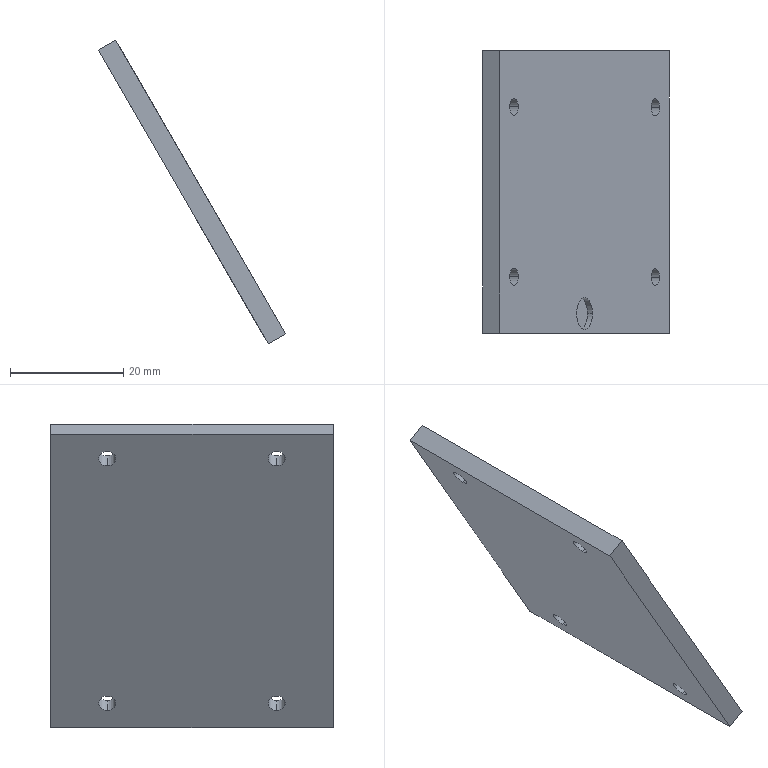Component | SolidWorks | LaserWorkingHeadCover(Upper)2-7 | 1 solid | 17 faces | box 33.03 x 50 x 53.71 mm | volume 10376 mm3 | cylinder 10 | plane 7 | commonest cylinder face diameters 3 x8 5.6 x2
build123d program:
from build123d import *

# Parameters (mm, degrees)
SKETCH1_2_W         = 60
SKETCH1_2_H         = 50
SKETCH1_2_R         = 1.5
BOSS_EXTRUDE1_DEPTH = 3.5
SKETCH1_R           = 2.8
CUT_EXTRUDE1_DEPTH  = 1


with BuildPart() as part:
    # Sketch1_2 → Boss-Extrude1 (new body)
    with BuildSketch(Plane.XY):
        Rectangle(SKETCH1_2_W, SKETCH1_2_H)
        with Locations((-25, 15)):
            Circle(SKETCH1_2_R, mode=Mode.SUBTRACT)
        with Locations((25, 15)):
            Circle(SKETCH1_2_R, mode=Mode.SUBTRACT)
        with Locations((25, -15)):
            Circle(SKETCH1_2_R, mode=Mode.SUBTRACT)
        with Locations((-25, -15)):
            Circle(SKETCH1_2_R, mode=Mode.SUBTRACT)
    extrude(amount=BOSS_EXTRUDE1_DEPTH)

    # Sketch1 → Cut-Extrude1 (cut)
    with BuildSketch(Plane(origin=(0, 0, 0), x_dir=(-1, 0, 0), z_dir=(0, 0, -1))):
        with Locations((0, -21.5)):
            Circle(SKETCH1_R)
    extrude(amount=-CUT_EXTRUDE1_DEPTH, mode=Mode.SUBTRACT)


solid = part.part

# Placed as in the assembly
solid = solid.moved(Location((-85.655, 40.506, 114), (-180, -60, 180)))
STEP:
#1=CARTESIAN_POINT('',(-3.461,0.7483,4.564));
#2=VERTEX_POINT('',#1);
#3=CARTESIAN_POINT('',(-3.351,0.7483,4.373));
#4=VERTEX_POINT('',#3);
#5=CARTESIAN_POINT('',(-3.406,0.7483,4.469));
#6=DIRECTION('',(0.866,-0.,0.5));
#7=DIRECTION('',(0.5,0.,-0.866));
#8=AXIS2_PLACEMENT_3D('',#5,#6,#7);
#9=CIRCLE('',#8,0.1102);
#10=EDGE_CURVE('',#2,#4,#9,.T.);
#11=ORIENTED_EDGE('',*,*,#10,.F.);
#12=CARTESIAN_POINT('',(-3.427,0.7483,4.584));
#13=VERTEX_POINT('',#12);
#14=CARTESIAN_POINT('',(-3.461,0.7483,4.564));
#15=DIRECTION('',(0.866,-0.,0.5));
#16=VECTOR('',#15,39.37);
#17=LINE('',#14,#16);
#18=EDGE_CURVE('',#2,#13,#17,.T.);
#19=ORIENTED_EDGE('',*,*,#18,.T.);
#20=CARTESIAN_POINT('',(-3.317,0.7483,4.393));
#21=VERTEX_POINT('',#20);
#22=CARTESIAN_POINT('',(-3.372,0.7483,4.488));
#23=DIRECTION('',(0.866,-0.,0.5));
#24=DIRECTION('',(0.5,0.,-0.866));
#25=AXIS2_PLACEMENT_3D('',#22,#23,#24);
#26=CIRCLE('',#25,0.1102);
#27=EDGE_CURVE('',#13,#21,#26,.T.);
#28=ORIENTED_EDGE('',*,*,#27,.T.);
#29=CARTESIAN_POINT('',(-3.351,0.7483,4.373));
#30=DIRECTION('',(0.866,-0.,0.5));
#31=VECTOR('',#30,39.37);
#32=LINE('',#29,#31);
#33=EDGE_CURVE('',#4,#21,#32,.T.);
#34=ORIENTED_EDGE('',*,*,#33,.F.);
#35=EDGE_LOOP('',(#11,#19,#28,#34));
#36=FACE_OUTER_BOUND('',#35,.T.);
#37=CARTESIAN_POINT('',(-3.406,0.7483,4.469));
#38=DIRECTION('',(0.866,-0.,0.5));
#39=DIRECTION('',(0.5,0.,-0.866));
#40=AXIS2_PLACEMENT_3D('',#37,#38,#39);
#41=CYLINDRICAL_SURFACE('',#40,0.1102);
#42=ADVANCED_FACE('',(#36),#41,.F.);
#43=CARTESIAN_POINT('',(-2.97,1.004,3.516));
#44=VERTEX_POINT('',#43);
#45=CARTESIAN_POINT('',(-3.029,1.004,3.618));
#46=VERTEX_POINT('',#45);
#47=CARTESIAN_POINT('',(-2.999,1.004,3.567));
#48=DIRECTION('',(-0.866,0.,-0.5));
#49=DIRECTION('',(-0.5,0.,0.866));
#50=AXIS2_PLACEMENT_3D('',#47,#48,#49);
#51=CIRCLE('',#50,0.05906);
#52=EDGE_CURVE('',#44,#46,#51,.T.);
#53=ORIENTED_EDGE('',*,*,#52,.T.);
#54=CARTESIAN_POINT('',(-2.91,1.004,3.687));
#55=VERTEX_POINT('',#54);
#56=CARTESIAN_POINT('',(-3.029,1.004,3.618));
#57=DIRECTION('',(0.866,-0.,0.5));
#58=VECTOR('',#57,39.37);
#59=LINE('',#56,#58);
#60=EDGE_CURVE('',#46,#55,#59,.T.);
#61=ORIENTED_EDGE('',*,*,#60,.T.);
#62=CARTESIAN_POINT('',(-2.851,1.004,3.585));
#63=VERTEX_POINT('',#62);
#64=CARTESIAN_POINT('',(-2.88,1.004,3.636));
#65=DIRECTION('',(-0.866,0.,-0.5));
#66=DIRECTION('',(-0.5,0.,0.866));
#67=AXIS2_PLACEMENT_3D('',#64,#65,#66);
#68=CIRCLE('',#67,0.05906);
#69=EDGE_CURVE('',#63,#55,#68,.T.);
#70=ORIENTED_EDGE('',*,*,#69,.F.);
#71=CARTESIAN_POINT('',(-2.97,1.004,3.516));
#72=DIRECTION('',(0.866,-0.,0.5));
#73=VECTOR('',#72,39.37);
#74=LINE('',#71,#73);
#75=EDGE_CURVE('',#44,#63,#74,.T.);
#76=ORIENTED_EDGE('',*,*,#75,.F.);
#77=EDGE_LOOP('',(#53,#61,#70,#76));
#78=FACE_OUTER_BOUND('',#77,.T.);
#79=CARTESIAN_POINT('',(-2.999,1.004,3.567));
#80=DIRECTION('',(0.866,-0.,0.5));
#81=DIRECTION('',(0.5,0.,-0.866));
#82=AXIS2_PLACEMENT_3D('',#79,#80,#81);
#83=CYLINDRICAL_SURFACE('',#82,0.05906);
#84=ADVANCED_FACE('',(#78),#83,.F.);
#85=CARTESIAN_POINT('',(-3.954,1.004,5.221));
#86=VERTEX_POINT('',#85);
#87=CARTESIAN_POINT('',(-4.013,1.004,5.323));
#88=VERTEX_POINT('',#87);
#89=CARTESIAN_POINT('',(-3.984,1.004,5.272));
#90=DIRECTION('',(-0.866,0.,-0.5));
#91=DIRECTION('',(-0.5,0.,0.866));
#92=AXIS2_PLACEMENT_3D('',#89,#90,#91);
#93=CIRCLE('',#92,0.05906);
#94=EDGE_CURVE('',#86,#88,#93,.T.);
#95=ORIENTED_EDGE('',*,*,#94,.T.);
#96=CARTESIAN_POINT('',(-3.894,1.004,5.392));
#97=VERTEX_POINT('',#96);
#98=CARTESIAN_POINT('',(-4.013,1.004,5.323));
#99=DIRECTION('',(0.866,-0.,0.5));
#100=VECTOR('',#99,39.37);
#101=LINE('',#98,#100);
#102=EDGE_CURVE('',#88,#97,#101,.T.);
#103=ORIENTED_EDGE('',*,*,#102,.T.);
#104=CARTESIAN_POINT('',(-3.835,1.004,5.289));
#105=VERTEX_POINT('',#104);
#106=CARTESIAN_POINT('',(-3.864,1.004,5.341));
#107=DIRECTION('',(-0.866,0.,-0.5));
#108=DIRECTION('',(-0.5,0.,0.866));
#109=AXIS2_PLACEMENT_3D('',#106,#107,#108);
#110=CIRCLE('',#109,0.05906);
#111=EDGE_CURVE('',#105,#97,#110,.T.);
#112=ORIENTED_EDGE('',*,*,#111,.F.);
#113=CARTESIAN_POINT('',(-3.954,1.004,5.221));
#114=DIRECTION('',(0.866,-0.,0.5));
#115=VECTOR('',#114,39.37);
#116=LINE('',#113,#115);
#117=EDGE_CURVE('',#86,#105,#116,.T.);
#118=ORIENTED_EDGE('',*,*,#117,.F.);
#119=EDGE_LOOP('',(#95,#103,#112,#118));
#120=FACE_OUTER_BOUND('',#119,.T.);
#121=CARTESIAN_POINT('',(-3.984,1.004,5.272));
#122=DIRECTION('',(0.866,-0.,0.5));
#123=DIRECTION('',(0.5,0.,-0.866));
#124=AXIS2_PLACEMENT_3D('',#121,#122,#123);
#125=CYLINDRICAL_SURFACE('',#124,0.05906);
#126=ADVANCED_FACE('',(#120),#125,.F.);
#127=CARTESIAN_POINT('',(-3.954,2.185,5.221));
#128=VERTEX_POINT('',#127);
#129=CARTESIAN_POINT('',(-4.013,2.185,5.323));
#130=VERTEX_POINT('',#129);
#131=CARTESIAN_POINT('',(-3.984,2.185,5.272));
#132=DIRECTION('',(-0.866,0.,-0.5));
#133=DIRECTION('',(-0.5,0.,0.866));
#134=AXIS2_PLACEMENT_3D('',#131,#132,#133);
#135=CIRCLE('',#134,0.05906);
#136=EDGE_CURVE('',#128,#130,#135,.T.);
#137=ORIENTED_EDGE('',*,*,#136,.T.);
#138=CARTESIAN_POINT('',(-3.894,2.185,5.392));
#139=VERTEX_POINT('',#138);
#140=CARTESIAN_POINT('',(-4.013,2.185,5.323));
#141=DIRECTION('',(0.866,-0.,0.5));
#142=VECTOR('',#141,39.37);
#143=LINE('',#140,#142);
#144=EDGE_CURVE('',#130,#139,#143,.T.);
#145=ORIENTED_EDGE('',*,*,#144,.T.);
#146=CARTESIAN_POINT('',(-3.835,2.185,5.289));
#147=VERTEX_POINT('',#146);
#148=CARTESIAN_POINT('',(-3.864,2.185,5.341));
#149=DIRECTION('',(-0.866,0.,-0.5));
#150=DIRECTION('',(-0.5,0.,0.866));
#151=AXIS2_PLACEMENT_3D('',#148,#149,#150);
#152=CIRCLE('',#151,0.05906);
#153=EDGE_CURVE('',#147,#139,#152,.T.);
#154=ORIENTED_EDGE('',*,*,#153,.F.);
#155=CARTESIAN_POINT('',(-3.954,2.185,5.221));
#156=DIRECTION('',(0.866,-0.,0.5));
#157=VECTOR('',#156,39.37);
#158=LINE('',#155,#157);
#159=EDGE_CURVE('',#128,#147,#158,.T.);
#160=ORIENTED_EDGE('',*,*,#159,.F.);
#161=EDGE_LOOP('',(#137,#145,#154,#160));
#162=FACE_OUTER_BOUND('',#161,.T.);
#163=CARTESIAN_POINT('',(-3.984,2.185,5.272));
#164=DIRECTION('',(0.866,-0.,0.5));
#165=DIRECTION('',(0.5,0.,-0.866));
#166=AXIS2_PLACEMENT_3D('',#163,#164,#165);
#167=CYLINDRICAL_SURFACE('',#166,0.05906);
#168=ADVANCED_FACE('',(#162),#167,.F.);
#169=CARTESIAN_POINT('',(-2.97,2.185,3.516));
#170=VERTEX_POINT('',#169);
#171=CARTESIAN_POINT('',(-3.029,2.185,3.618));
#172=VERTEX_POINT('',#171);
#173=CARTESIAN_POINT('',(-2.999,2.185,3.567));
#174=DIRECTION('',(-0.866,0.,-0.5));
#175=DIRECTION('',(-0.5,0.,0.866));
#176=AXIS2_PLACEMENT_3D('',#173,#174,#175);
#177=CIRCLE('',#176,0.05906);
#178=EDGE_CURVE('',#170,#172,#177,.T.);
#179=ORIENTED_EDGE('',*,*,#178,.T.);
#180=CARTESIAN_POINT('',(-2.91,2.185,3.687));
#181=VERTEX_POINT('',#180);
#182=CARTESIAN_POINT('',(-3.029,2.185,3.618));
#183=DIRECTION('',(0.866,-0.,0.5));
#184=VECTOR('',#183,39.37);
#185=LINE('',#182,#184);
#186=EDGE_CURVE('',#172,#181,#185,.T.);
#187=ORIENTED_EDGE('',*,*,#186,.T.);
#188=CARTESIAN_POINT('',(-2.851,2.185,3.585));
#189=VERTEX_POINT('',#188);
#190=CARTESIAN_POINT('',(-2.88,2.185,3.636));
#191=DIRECTION('',(-0.866,0.,-0.5));
#192=DIRECTION('',(-0.5,0.,0.866));
#193=AXIS2_PLACEMENT_3D('',#190,#191,#192);
#194=CIRCLE('',#193,0.05906);
#195=EDGE_CURVE('',#189,#181,#194,.T.);
#196=ORIENTED_EDGE('',*,*,#195,.F.);
#197=CARTESIAN_POINT('',(-2.97,2.185,3.516));
#198=DIRECTION('',(0.866,-0.,0.5));
#199=VECTOR('',#198,39.37);
#200=LINE('',#197,#199);
#201=EDGE_CURVE('',#170,#189,#200,.T.);
#202=ORIENTED_EDGE('',*,*,#201,.F.);
#203=EDGE_LOOP('',(#179,#187,#196,#202));
#204=FACE_OUTER_BOUND('',#203,.T.);
#205=CARTESIAN_POINT('',(-2.999,2.185,3.567));
#206=DIRECTION('',(0.866,-0.,0.5));
#207=DIRECTION('',(0.5,0.,-0.866));
#208=AXIS2_PLACEMENT_3D('',#205,#206,#207);
#209=CYLINDRICAL_SURFACE('',#208,0.05906);
#210=ADVANCED_FACE('',(#204),#209,.F.);
#211=ORIENTED_EDGE('',*,*,#94,.F.);
#212=CARTESIAN_POINT('',(-3.984,1.004,5.272));
#213=DIRECTION('',(-0.866,0.,-0.5));
#214=DIRECTION('',(-0.5,0.,0.866));
#215=AXIS2_PLACEMENT_3D('',#212,#213,#214);
#216=CIRCLE('',#215,0.05906);
#217=EDGE_CURVE('',#88,#86,#216,.T.);
#218=ORIENTED_EDGE('',*,*,#217,.F.);
#219=EDGE_LOOP('',(#211,#218));
#220=FACE_BOUND('',#219,.T.);
#221=ORIENTED_EDGE('',*,*,#178,.F.);
#222=CARTESIAN_POINT('',(-2.999,2.185,3.567));
#223=DIRECTION('',(-0.866,0.,-0.5));
#224=DIRECTION('',(-0.5,0.,0.866));
#225=AXIS2_PLACEMENT_3D('',#222,#223,#224);
#226=CIRCLE('',#225,0.05906);
#227=EDGE_CURVE('',#172,#170,#226,.T.);
#228=ORIENTED_EDGE('',*,*,#227,.F.);
#229=EDGE_LOOP('',(#221,#228));
#230=FACE_BOUND('',#229,.T.);
#231=CARTESIAN_POINT('',(-4.082,0.6105,5.442));
#232=VERTEX_POINT('',#231);
#233=CARTESIAN_POINT('',(-4.082,2.579,5.442));
#234=VERTEX_POINT('',#233);
#235=CARTESIAN_POINT('',(-4.082,2.579,5.442));
#236=DIRECTION('',(0.,1.,-0.));
#237=VECTOR('',#236,39.37);
#238=LINE('',#235,#237);
#239=EDGE_CURVE('',#232,#234,#238,.T.);
#240=ORIENTED_EDGE('',*,*,#239,.T.);
#241=CARTESIAN_POINT('',(-2.901,2.579,3.396));
#242=VERTEX_POINT('',#241);
#243=CARTESIAN_POINT('',(-2.901,2.579,3.396));
#244=DIRECTION('',(0.5,-0.,-0.866));
#245=VECTOR('',#244,39.37);
#246=LINE('',#243,#245);
#247=EDGE_CURVE('',#234,#242,#246,.T.);
#248=ORIENTED_EDGE('',*,*,#247,.T.);
#249=CARTESIAN_POINT('',(-2.901,0.6105,3.396));
#250=VERTEX_POINT('',#249);
#251=CARTESIAN_POINT('',(-2.901,2.579,3.396));
#252=DIRECTION('',(-0.,-1.,0.));
#253=VECTOR('',#252,39.37);
#254=LINE('',#251,#253);
#255=EDGE_CURVE('',#242,#250,#254,.T.);
#256=ORIENTED_EDGE('',*,*,#255,.T.);
#257=CARTESIAN_POINT('',(-2.901,0.6105,3.396));
#258=DIRECTION('',(-0.5,0.,0.866));
#259=VECTOR('',#258,39.37);
#260=LINE('',#257,#259);
#261=EDGE_CURVE('',#250,#232,#260,.T.);
#262=ORIENTED_EDGE('',*,*,#261,.T.);
#263=EDGE_LOOP('',(#240,#248,#256,#262));
#264=FACE_OUTER_BOUND('',#263,.T.);
#265=ORIENTED_EDGE('',*,*,#136,.F.);
#266=CARTESIAN_POINT('',(-3.984,2.185,5.272));
#267=DIRECTION('',(-0.866,0.,-0.5));
#268=DIRECTION('',(-0.5,0.,0.866));
#269=AXIS2_PLACEMENT_3D('',#266,#267,#268);
#270=CIRCLE('',#269,0.05906);
#271=EDGE_CURVE('',#130,#128,#270,.T.);
#272=ORIENTED_EDGE('',*,*,#271,.F.);
#273=EDGE_LOOP('',(#265,#272));
#274=FACE_BOUND('',#273,.T.);
#275=ORIENTED_EDGE('',*,*,#52,.F.);
#276=CARTESIAN_POINT('',(-2.999,1.004,3.567));
#277=DIRECTION('',(-0.866,0.,-0.5));
#278=DIRECTION('',(-0.5,0.,0.866));
#279=AXIS2_PLACEMENT_3D('',#276,#277,#278);
#280=CIRCLE('',#279,0.05906);
#281=EDGE_CURVE('',#46,#44,#280,.T.);
#282=ORIENTED_EDGE('',*,*,#281,.F.);
#283=EDGE_LOOP('',(#275,#282));
#284=FACE_BOUND('',#283,.T.);
#285=CARTESIAN_POINT('',(-3.492,1.595,4.419));
#286=DIRECTION('',(-0.866,0.,-0.5));
#287=DIRECTION('',(-0.5,0.,0.866));
#288=AXIS2_PLACEMENT_3D('',#285,#286,#287);
#289=PLANE('',#288);
#290=ADVANCED_FACE('',(#220,#230,#264,#274,#284),#289,.T.);
#291=CARTESIAN_POINT('',(-3.372,0.7483,4.488));
#292=DIRECTION('',(0.866,-0.,0.5));
#293=DIRECTION('',(0.5,0.,-0.866));
#294=AXIS2_PLACEMENT_3D('',#291,#292,#293);
#295=CIRCLE('',#294,0.1102);
#296=EDGE_CURVE('',#21,#13,#295,.T.);
#297=ORIENTED_EDGE('',*,*,#296,.F.);
#298=ORIENTED_EDGE('',*,*,#27,.F.);
#299=EDGE_LOOP('',(#297,#298));
#300=FACE_BOUND('',#299,.T.);
#301=CARTESIAN_POINT('',(-3.963,0.6105,5.511));
#302=VERTEX_POINT('',#301);
#303=CARTESIAN_POINT('',(-3.963,2.579,5.511));
#304=VERTEX_POINT('',#303);
#305=CARTESIAN_POINT('',(-3.963,2.579,5.511));
#306=DIRECTION('',(0.,1.,-0.));
#307=VECTOR('',#306,39.37);
#308=LINE('',#305,#307);
#309=EDGE_CURVE('',#302,#304,#308,.T.);
#310=ORIENTED_EDGE('',*,*,#309,.F.);
#311=CARTESIAN_POINT('',(-2.782,0.6105,3.465));
#312=VERTEX_POINT('',#311);
#313=CARTESIAN_POINT('',(-2.782,0.6105,3.465));
#314=DIRECTION('',(-0.5,0.,0.866));
#315=VECTOR('',#314,39.37);
#316=LINE('',#313,#315);
#317=EDGE_CURVE('',#312,#302,#316,.T.);
#318=ORIENTED_EDGE('',*,*,#317,.F.);
#319=CARTESIAN_POINT('',(-2.782,2.579,3.465));
#320=VERTEX_POINT('',#319);
#321=CARTESIAN_POINT('',(-2.782,2.579,3.465));
#322=DIRECTION('',(-0.,-1.,0.));
#323=VECTOR('',#322,39.37);
#324=LINE('',#321,#323);
#325=EDGE_CURVE('',#320,#312,#324,.T.);
#326=ORIENTED_EDGE('',*,*,#325,.F.);
#327=CARTESIAN_POINT('',(-2.782,2.579,3.465));
#328=DIRECTION('',(0.5,-0.,-0.866));
#329=VECTOR('',#328,39.37);
#330=LINE('',#327,#329);
#331=EDGE_CURVE('',#304,#320,#330,.T.);
#332=ORIENTED_EDGE('',*,*,#331,.F.);
#333=EDGE_LOOP('',(#310,#318,#326,#332));
#334=FACE_OUTER_BOUND('',#333,.T.);
#335=ORIENTED_EDGE('',*,*,#195,.T.);
#336=CARTESIAN_POINT('',(-2.88,2.185,3.636));
#337=DIRECTION('',(-0.866,0.,-0.5));
#338=DIRECTION('',(-0.5,0.,0.866));
#339=AXIS2_PLACEMENT_3D('',#336,#337,#338);
#340=CIRCLE('',#339,0.05906);
#341=EDGE_CURVE('',#181,#189,#340,.T.);
#342=ORIENTED_EDGE('',*,*,#341,.T.);
#343=EDGE_LOOP('',(#335,#342));
#344=FACE_BOUND('',#343,.T.);
#345=ORIENTED_EDGE('',*,*,#153,.T.);
#346=CARTESIAN_POINT('',(-3.864,2.185,5.341));
#347=DIRECTION('',(-0.866,0.,-0.5));
#348=DIRECTION('',(-0.5,0.,0.866));
#349=AXIS2_PLACEMENT_3D('',#346,#347,#348);
#350=CIRCLE('',#349,0.05906);
#351=EDGE_CURVE('',#139,#147,#350,.T.);
#352=ORIENTED_EDGE('',*,*,#351,.T.);
#353=EDGE_LOOP('',(#345,#352));
#354=FACE_BOUND('',#353,.T.);
#355=ORIENTED_EDGE('',*,*,#111,.T.);
#356=CARTESIAN_POINT('',(-3.864,1.004,5.341));
#357=DIRECTION('',(-0.866,0.,-0.5));
#358=DIRECTION('',(-0.5,0.,0.866));
#359=AXIS2_PLACEMENT_3D('',#356,#357,#358);
#360=CIRCLE('',#359,0.05906);
#361=EDGE_CURVE('',#97,#105,#360,.T.);
#362=ORIENTED_EDGE('',*,*,#361,.T.);
#363=EDGE_LOOP('',(#355,#362));
#364=FACE_BOUND('',#363,.T.);
#365=ORIENTED_EDGE('',*,*,#69,.T.);
#366=CARTESIAN_POINT('',(-2.88,1.004,3.636));
#367=DIRECTION('',(-0.866,0.,-0.5));
#368=DIRECTION('',(-0.5,0.,0.866));
#369=AXIS2_PLACEMENT_3D('',#366,#367,#368);
#370=CIRCLE('',#369,0.05906);
#371=EDGE_CURVE('',#55,#63,#370,.T.);
#372=ORIENTED_EDGE('',*,*,#371,.T.);
#373=EDGE_LOOP('',(#365,#372));
#374=FACE_BOUND('',#373,.T.);
#375=CARTESIAN_POINT('',(-3.372,1.595,4.488));
#376=DIRECTION('',(-0.866,0.,-0.5));
#377=DIRECTION('',(-0.5,0.,0.866));
#378=AXIS2_PLACEMENT_3D('',#375,#376,#377);
#379=PLANE('',#378);
#380=ADVANCED_FACE('',(#300,#334,#344,#354,#364,#374),#379,.F.);
#381=ORIENTED_EDGE('',*,*,#309,.T.);
#382=CARTESIAN_POINT('',(-4.082,2.579,5.442));
#383=DIRECTION('',(0.866,-0.,0.5));
#384=VECTOR('',#383,39.37);
#385=LINE('',#382,#384);
#386=EDGE_CURVE('',#234,#304,#385,.T.);
#387=ORIENTED_EDGE('',*,*,#386,.F.);
#388=ORIENTED_EDGE('',*,*,#239,.F.);
#389=CARTESIAN_POINT('',(-4.082,0.6105,5.442));
#390=DIRECTION('',(0.866,-0.,0.5));
#391=VECTOR('',#390,39.37);
#392=LINE('',#389,#391);
#393=EDGE_CURVE('',#232,#302,#392,.T.);
#394=ORIENTED_EDGE('',*,*,#393,.T.);
#395=EDGE_LOOP('',(#381,#387,#388,#394));
#396=FACE_OUTER_BOUND('',#395,.T.);
#397=CARTESIAN_POINT('',(-4.082,2.579,5.442));
#398=DIRECTION('',(0.5,-0.,-0.866));
#399=DIRECTION('',(-0.866,0.,-0.5));
#400=AXIS2_PLACEMENT_3D('',#397,#398,#399);
#401=PLANE('',#400);
#402=ADVANCED_FACE('',(#396),#401,.F.);
#403=ORIENTED_EDGE('',*,*,#331,.T.);
#404=CARTESIAN_POINT('',(-2.901,2.579,3.396));
#405=DIRECTION('',(0.866,-0.,0.5));
#406=VECTOR('',#405,39.37);
#407=LINE('',#404,#406);
#408=EDGE_CURVE('',#242,#320,#407,.T.);
#409=ORIENTED_EDGE('',*,*,#408,.F.);
#410=ORIENTED_EDGE('',*,*,#247,.F.);
#411=ORIENTED_EDGE('',*,*,#386,.T.);
#412=EDGE_LOOP('',(#403,#409,#410,#411));
#413=FACE_OUTER_BOUND('',#412,.T.);
#414=CARTESIAN_POINT('',(-2.901,2.579,3.396));
#415=DIRECTION('',(-0.,-1.,0.));
#416=DIRECTION('',(0.866,-0.,0.5));
#417=AXIS2_PLACEMENT_3D('',#414,#415,#416);
#418=PLANE('',#417);
#419=ADVANCED_FACE('',(#413),#418,.F.);
#420=ORIENTED_EDGE('',*,*,#325,.T.);
#421=CARTESIAN_POINT('',(-2.901,0.6105,3.396));
#422=DIRECTION('',(0.866,-0.,0.5));
#423=VECTOR('',#422,39.37);
#424=LINE('',#421,#423);
#425=EDGE_CURVE('',#250,#312,#424,.T.);
#426=ORIENTED_EDGE('',*,*,#425,.F.);
#427=ORIENTED_EDGE('',*,*,#255,.F.);
#428=ORIENTED_EDGE('',*,*,#408,.T.);
#429=EDGE_LOOP('',(#420,#426,#427,#428));
#430=FACE_OUTER_BOUND('',#429,.T.);
#431=CARTESIAN_POINT('',(-2.901,2.579,3.396));
#432=DIRECTION('',(-0.5,0.,0.866));
#433=DIRECTION('',(0.,1.,-0.));
#434=AXIS2_PLACEMENT_3D('',#431,#432,#433);
#435=PLANE('',#434);
#436=ADVANCED_FACE('',(#430),#435,.F.);
#437=ORIENTED_EDGE('',*,*,#317,.T.);
#438=ORIENTED_EDGE('',*,*,#393,.F.);
#439=ORIENTED_EDGE('',*,*,#261,.F.);
#440=ORIENTED_EDGE('',*,*,#425,.T.);
#441=EDGE_LOOP('',(#437,#438,#439,#440));
#442=FACE_OUTER_BOUND('',#441,.T.);
#443=CARTESIAN_POINT('',(-2.901,0.6105,3.396));
#444=DIRECTION('',(0.,1.,-0.));
#445=DIRECTION('',(-0.866,0.,-0.5));
#446=AXIS2_PLACEMENT_3D('',#443,#444,#445);
#447=PLANE('',#446);
#448=ADVANCED_FACE('',(#442),#447,.F.);
#449=ORIENTED_EDGE('',*,*,#186,.F.);
#450=ORIENTED_EDGE('',*,*,#227,.T.);
#451=ORIENTED_EDGE('',*,*,#201,.T.);
#452=ORIENTED_EDGE('',*,*,#341,.F.);
#453=EDGE_LOOP('',(#449,#450,#451,#452));
#454=FACE_OUTER_BOUND('',#453,.T.);
#455=CARTESIAN_POINT('',(-2.999,2.185,3.567));
#456=DIRECTION('',(0.866,-0.,0.5));
#457=DIRECTION('',(0.5,0.,-0.866));
#458=AXIS2_PLACEMENT_3D('',#455,#456,#457);
#459=CYLINDRICAL_SURFACE('',#458,0.05906);
#460=ADVANCED_FACE('',(#454),#459,.F.);
#461=ORIENTED_EDGE('',*,*,#144,.F.);
#462=ORIENTED_EDGE('',*,*,#271,.T.);
#463=ORIENTED_EDGE('',*,*,#159,.T.);
#464=ORIENTED_EDGE('',*,*,#351,.F.);
#465=EDGE_LOOP('',(#461,#462,#463,#464));
#466=FACE_OUTER_BOUND('',#465,.T.);
#467=CARTESIAN_POINT('',(-3.984,2.185,5.272));
#468=DIRECTION('',(0.866,-0.,0.5));
#469=DIRECTION('',(0.5,0.,-0.866));
#470=AXIS2_PLACEMENT_3D('',#467,#468,#469);
#471=CYLINDRICAL_SURFACE('',#470,0.05906);
#472=ADVANCED_FACE('',(#466),#471,.F.);
#473=ORIENTED_EDGE('',*,*,#102,.F.);
#474=ORIENTED_EDGE('',*,*,#217,.T.);
#475=ORIENTED_EDGE('',*,*,#117,.T.);
#476=ORIENTED_EDGE('',*,*,#361,.F.);
#477=EDGE_LOOP('',(#473,#474,#475,#476));
#478=FACE_OUTER_BOUND('',#477,.T.);
#479=CARTESIAN_POINT('',(-3.984,1.004,5.272));
#480=DIRECTION('',(0.866,-0.,0.5));
#481=DIRECTION('',(0.5,0.,-0.866));
#482=AXIS2_PLACEMENT_3D('',#479,#480,#481);
#483=CYLINDRICAL_SURFACE('',#482,0.05906);
#484=ADVANCED_FACE('',(#478),#483,.F.);
#485=ORIENTED_EDGE('',*,*,#60,.F.);
#486=ORIENTED_EDGE('',*,*,#281,.T.);
#487=ORIENTED_EDGE('',*,*,#75,.T.);
#488=ORIENTED_EDGE('',*,*,#371,.F.);
#489=EDGE_LOOP('',(#485,#486,#487,#488));
#490=FACE_OUTER_BOUND('',#489,.T.);
#491=CARTESIAN_POINT('',(-2.999,1.004,3.567));
#492=DIRECTION('',(0.866,-0.,0.5));
#493=DIRECTION('',(0.5,0.,-0.866));
#494=AXIS2_PLACEMENT_3D('',#491,#492,#493);
#495=CYLINDRICAL_SURFACE('',#494,0.05906);
#496=ADVANCED_FACE('',(#490),#495,.F.);
#497=ORIENTED_EDGE('',*,*,#18,.F.);
#498=CARTESIAN_POINT('',(-3.406,0.7483,4.469));
#499=DIRECTION('',(0.866,-0.,0.5));
#500=DIRECTION('',(0.5,0.,-0.866));
#501=AXIS2_PLACEMENT_3D('',#498,#499,#500);
#502=CIRCLE('',#501,0.1102);
#503=EDGE_CURVE('',#4,#2,#502,.T.);
#504=ORIENTED_EDGE('',*,*,#503,.F.);
#505=ORIENTED_EDGE('',*,*,#33,.T.);
#506=ORIENTED_EDGE('',*,*,#296,.T.);
#507=EDGE_LOOP('',(#497,#504,#505,#506));
#508=FACE_OUTER_BOUND('',#507,.T.);
#509=CARTESIAN_POINT('',(-3.406,0.7483,4.469));
#510=DIRECTION('',(0.866,-0.,0.5));
#511=DIRECTION('',(0.5,0.,-0.866));
#512=AXIS2_PLACEMENT_3D('',#509,#510,#511);
#513=CYLINDRICAL_SURFACE('',#512,0.1102);
#514=ADVANCED_FACE('',(#508),#513,.F.);
#515=ORIENTED_EDGE('',*,*,#503,.T.);
#516=ORIENTED_EDGE('',*,*,#10,.T.);
#517=EDGE_LOOP('',(#515,#516));
#518=FACE_OUTER_BOUND('',#517,.T.);
#519=CARTESIAN_POINT('',(-3.406,0.7483,4.469));
#520=DIRECTION('',(0.866,-0.,0.5));
#521=DIRECTION('',(0.5,-0.,-0.866));
#522=AXIS2_PLACEMENT_3D('',#519,#520,#521);
#523=PLANE('',#522);
#524=ADVANCED_FACE('',(#518),#523,.T.);
#525=CLOSED_SHELL('',(#42,#84,#126,#168,#210,#290,#380,#402,#419,#436,#448,#460,#472,#484,#496,#514,#524));
#526=MANIFOLD_SOLID_BREP('',#525);
#527=CARTESIAN_POINT('',(0.,0.,0.));
#528=DIRECTION('',(0.,0.,1.));
#529=DIRECTION('',(1.,0.,0.));
#530=AXIS2_PLACEMENT_3D('',#527,#528,#529);
#531=(LENGTH_UNIT()NAMED_UNIT(*)SI_UNIT($,.METRE.));
#532=LENGTH_MEASURE_WITH_UNIT(LENGTH_MEASURE(0.0254),#531);
#533=DIMENSIONAL_EXPONENTS(1.,0.,0.,0.,0.,0.,0.);
#534=(CONVERSION_BASED_UNIT('',#532)LENGTH_UNIT()NAMED_UNIT(#533));
#535=UNCERTAINTY_MEASURE_WITH_UNIT(LENGTH_MEASURE(0.00001),#534,'','');
#536=(NAMED_UNIT(*)PLANE_ANGLE_UNIT()SI_UNIT($,.RADIAN.));
#537=(NAMED_UNIT(*)SI_UNIT($,.STERADIAN.)SOLID_ANGLE_UNIT());
#538=(GEOMETRIC_REPRESENTATION_CONTEXT(3)GLOBAL_UNCERTAINTY_ASSIGNED_CONTEXT((#535))GLOBAL_UNIT_ASSIGNED_CONTEXT((#534,#536,#537))REPRESENTATION_CONTEXT('',''));
#539=ADVANCED_BREP_SHAPE_REPRESENTATION('',(#526,#530),#538);
#540=COLOUR_RGB('',0.7922,0.8196,0.9333);
#541=FILL_AREA_STYLE_COLOUR('',#540);
#542=FILL_AREA_STYLE('',(#541));
#543=SURFACE_STYLE_FILL_AREA(#542);
#544=SURFACE_SIDE_STYLE('',(#543));
#545=SURFACE_STYLE_USAGE(.BOTH.,#544);
#546=PRESENTATION_STYLE_ASSIGNMENT((#545));
#547=STYLED_ITEM('',(#546),#526);
#548=PRESENTATION_LAYER_ASSIGNMENT('','',(#547));
#549=(LENGTH_UNIT()NAMED_UNIT(*)SI_UNIT($,.METRE.));
#550=LENGTH_MEASURE_WITH_UNIT(LENGTH_MEASURE(0.0254),#549);
#551=DIMENSIONAL_EXPONENTS(1.,0.,0.,0.,0.,0.,0.);
#552=(CONVERSION_BASED_UNIT('',#550)LENGTH_UNIT()NAMED_UNIT(#551));
#553=UNCERTAINTY_MEASURE_WITH_UNIT(LENGTH_MEASURE(0.00001),#552,'','');
#554=(NAMED_UNIT(*)PLANE_ANGLE_UNIT()SI_UNIT($,.RADIAN.));
#555=(NAMED_UNIT(*)SI_UNIT($,.STERADIAN.)SOLID_ANGLE_UNIT());
#556=(GEOMETRIC_REPRESENTATION_CONTEXT(3)GLOBAL_UNCERTAINTY_ASSIGNED_CONTEXT((#553))GLOBAL_UNIT_ASSIGNED_CONTEXT((#552,#554,#555))REPRESENTATION_CONTEXT('',''));
#557=MECHANICAL_DESIGN_GEOMETRIC_PRESENTATION_REPRESENTATION('',(#547),#556);